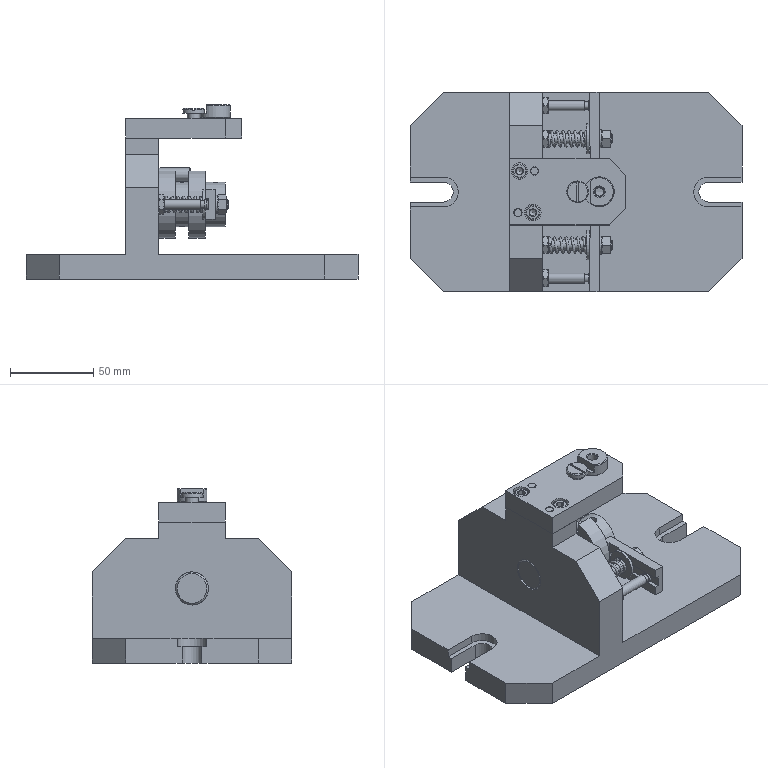Assembly | NX | mm | 30 component files | 30 solids | 481 faces | box 200 x 120 x 105 mm | volume 558934 mm3 | plane 233 | cone 139 | cylinder 93 | spline 10 | torus 4 | sphere 2 | commonest cylinder face diameters 6 x19 5 x13 5.188 x12 18 x5 10 x4 6.4 x4 6.6 x4 20 x4
Bill of materials:
GB-T6172_1-2000,M6x1 | 4 |  | Hexagon Thin Nut, Chamfered, GB-T 6172.1-2000,M6x1
unnamed part 1 | 1 |  | Hollow cylindrical sleeve with two raised outer collars. Each collar has a rectangular notch, and the two notches line up axially. Small radial holes pass through the smaller-diameter sections.
unnamed part 2 | 1 |  | Stepped, rotationally symmetric pin with a slotted round head. Below the head, in order: a cylindrical shoulder, a reduced-diameter neck, and a chamfered cylindrical end section.
GB-T70.1-2000,M5x12 | 2 |  | Hexagon Socket Head Cap Screw, GB-T 70.1-2000,M5x12
GB-T848-2002,M6 | 2 |  | Flat annular ring (washer-like disc) with a concentric through-hole; relatively large bore and moderately thick wall compared with its outer diameter.
GB-T6170_F-2000,M6x1 | 2 |  | Hexagonal prism with a central round through-hole. The corners are chamfered on both faces and the bore edge is chamfered, which is consistent with a hex-nut shape.
unnamed part 3 | 2 |  | Flat rectangular bar with an obround (slot-shaped) through-hole near one end. A shallow rectangular groove crosses one face near the other end.
unnamed part 4 | 1 |  | Stepped cylindrical part with a central through-hole. It has a large round head, a reduced neck, and a chamfered cylindrical shank. Part of the head's height is cut away on one side, leaving a stepped region.
GB-T119.1-2000,5x22 | 2 |  | Parallel Pin, GB-T 119.1-2000,5x22
GB-T96_1-2002,M6 | 2 |  | Thin flat annular disc (washer-like) with a small concentric through-hole and a wide flat face.
unnamed part 5 | 1 |  | Solid cylindrical pin with an integral central collar. Reduced-diameter necks sit on both sides of the collar, followed by two chamfered cylindrical end sections of different lengths.
unnamed part 6 | 1 |  | Plain cylindrical tube or bushing shape with a through-bore. The inner and outer edges at both ends are chamfered.
unnamed part 7 | 2 |  | Helical coil of round wire with roughly seven to eight turns and constant diameter and pitch. Each end is cut to a flat annular face, which is consistent with a coil-spring shape.
unnamed part 8 | 2 |  | Long, slender, solid cylindrical shaft with chamfered ends. Each end has a reduced-diameter groove or neck: one is set inward from the end, the other sits close to it.
unnamed part 9 | 1 |  | Solid stepped cylindrical pin with two diameters: a short, smaller-diameter section and a longer, larger-diameter section. The ends and the step are chamfered.
unnamed part 10 | 1 |  | Flat rectangular plate with two chamfered corners at one end. It has one large through-hole near the chamfered end, a small blind drilled hole beside it, and four smaller through-holes in two pairs near the opposite end.
unnamed part 11 | 1 |  | Bracket-like body: a rectangular base plate with chamfered corners and an open-ended U-slot at each short end, and an integral upright wall forming a T-shaped cross-section. The wall has a central large through-hole, several small blind holes, chamfered upper corners, and a raised rectangular top boss with four small holes.
unnamed part 12 | 2 |  | Solid, straight cylindrical pin with a single nominal outer diameter. It has two circumferential grooves. The first is wider and shallow, located about one-fifth of the length from the flat end. The second is narrower and deeper, located just behind a short domed (rounded) tip at the other end. The flat end is plain.
Mates:
1. concentric | mandrel 1 edge | fixture_body 1 edge
2. concentric | stop_block_wp 1 edge | mandrel 1 edge
3. concentric | loc_pin 1 edge | fixture_body 1 arc
4. touch align | clamp_plate 2 face | fixture_body 1 face
5. touch align | clamp_plate 2 face | stop_block_wp 1 face
6. distance | fix_stud 2 face | fixture_body 1 face
7. touch align | fix_stud 2 face | fixture_body 1 face
8. touch align | support_stud 2 face | fixture_body 1 face
9. distance | support_stud 2 face | fixture_body 1 face
10. concentric | GB-T6172_1-2000_M6x1 4 edge | fixture_body 1 arc
11. concentric | GB-T6172_1-2000_M6x1 3 edge | fixture_body 1 arc
12. touch align | GB-T96_1-2002_M6 2 face | fix_stud 2 face
13. touch align | GB-T96_1-2002_M6 2 face | clamp_plate 2 face
14. concentric | spring 2 edge | GB-T6172_1-2000_M6x1 4 edge
15. concentric | GB-T848-2002_M6 2 edge | clamp_plate 2 edge
16. concentric | GB-T6170_F-2000_M6x1 2 edge | GB-T848-2002_M6 2 edge
17. bond | stop_block_wp 1 component | assembly component
18. bond | clamp_plate 2 component | assembly component
19. bond | support_stud 2 component | assembly component
20. bond | GB-T6172_1-2000_M6x1 4 component | assembly component
21. bond | GB-T6172_1-2000_M6x1 3 component | assembly component
22. bond | GB-T96_1-2002_M6 2 component | assembly component
23. bond | spring 2 component | assembly component
24. bond | GB-T848-2002_M6 2 component | assembly component
25. bond | GB-T6170_F-2000_M6x1 2 component | assembly component
26. bond | clamp_plate 1 component | assembly component
27. bond | support_stud 1 component | assembly component
28. bond | GB-T6172_1-2000_M6x1 2 component | assembly component
29. bond | GB-T6172_1-2000_M6x1 1 component | assembly component
30. bond | GB-T96_1-2002_M6 1 component | assembly component
31. bond | spring 1 component | assembly component
32. bond | GB-T848-2002_M6 1 component | assembly component
33. bond | GB-T6170_F-2000_M6x1 1 component | assembly component
34. circular | assembly datumaxis | assembly cartesiancoordinatesystem | assembly cartesiancoordinatesystem
35. circular | assembly datumaxis | assembly cartesiancoordinatesystem | assembly cartesiancoordinatesystem
36. circular | assembly datumaxis | assembly cartesiancoordinatesystem | assembly cartesiancoordinatesystem
37. circular | assembly datumaxis | assembly cartesiancoordinatesystem | assembly cartesiancoordinatesystem
38. circular | assembly datumaxis | assembly cartesiancoordinatesystem | assembly cartesiancoordinatesystem
39. circular | assembly datumaxis | assembly cartesiancoordinatesystem | assembly cartesiancoordinatesystem
40. circular | assembly datumaxis | assembly cartesiancoordinatesystem | assembly cartesiancoordinatesystem
41. circular | assembly datumaxis | assembly cartesiancoordinatesystem | assembly cartesiancoordinatesystem
42. bond | fix_stud 2 component | assembly component
43. bond | fix_stud 1 component | assembly component
44. circular | assembly datumaxis | assembly cartesiancoordinatesystem | assembly cartesiancoordinatesystem
45. touch align | drill_template 1 face | fixture_body 1 face
46. touch align | drill_template 1 face | fixture_body 1 face
47. touch align | drill_template 1 face | fixture_body 1 face
48. concentric | bushing 1 edge | drill_template 1 edge
49. concentric | drill_bush 1 edge | bushing 1 edge
50. concentric | drill_bush_screw 1 edge | drill_template 1 arc